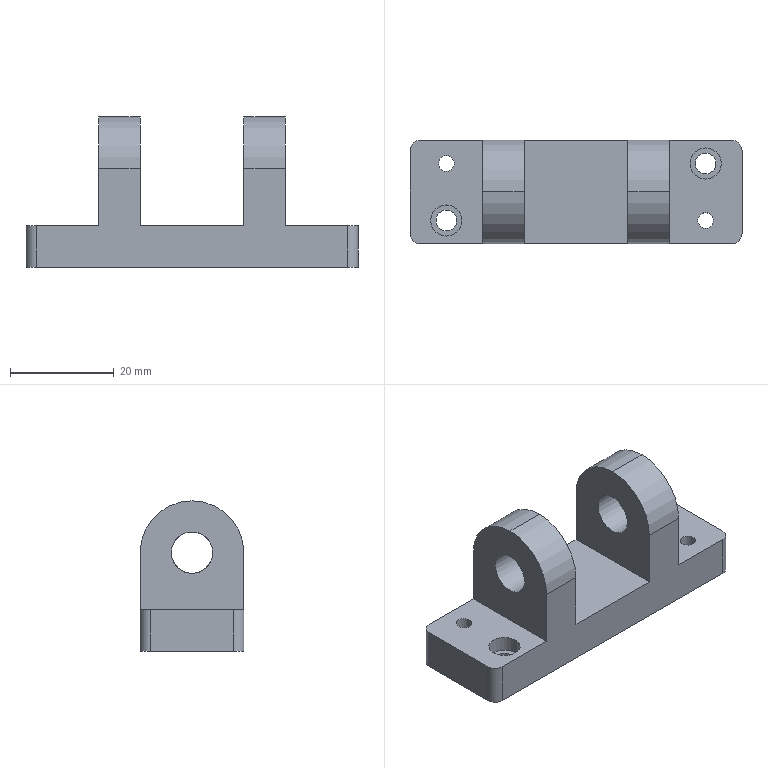Component | NX | BRACKET | 1 solid | 30 faces | volume 15033 mm3 | cylinder 16 | plane 14 | commonest cylinder face diameters 4 x6 20 x4 8 x2 3 x2 6 x2